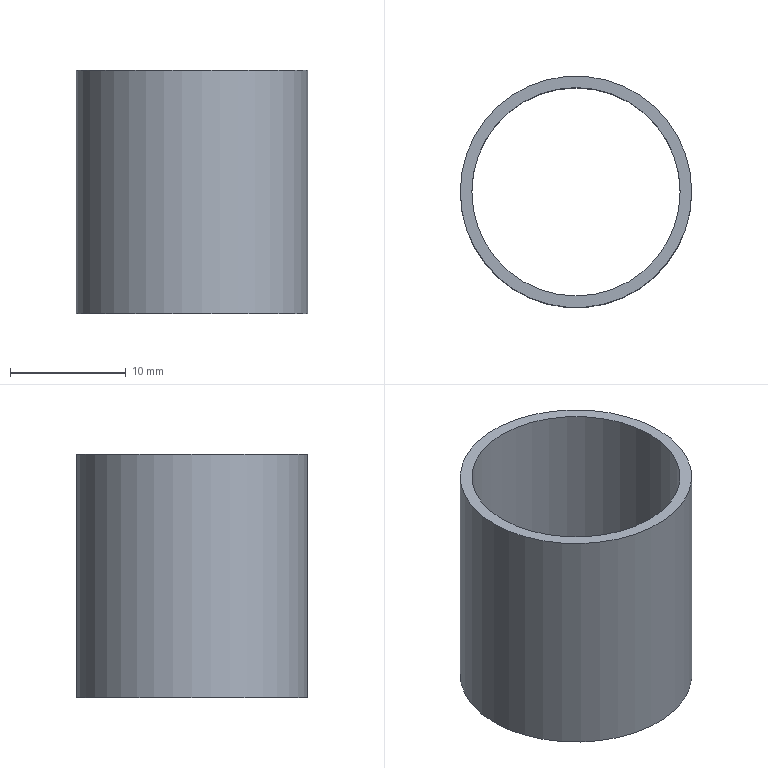Component | NX | 7_2 | 1 solid | 4 faces | box 20 x 20 x 21 mm | volume 1253 mm3 | cylinder 2 | plane 2 | commonest cylinder face diameters 20 x1 18 x1
STEP:
#1=CARTESIAN_POINT('',(0.,0.,0.));
#2=DIRECTION('',(0.,0.,1.));
#3=DIRECTION('',(1.,0.,0.));
#4=AXIS2_PLACEMENT_3D('',#1,#2,#3);
#5=CARTESIAN_POINT('',(10.,-16.5,29.));
#6=VERTEX_POINT('',#5);
#7=CARTESIAN_POINT('',(-0.0000016,-16.5,29.));
#8=DIRECTION('',(0.,0.,1.));
#9=DIRECTION('',(1.,0.00000005,0.));
#10=AXIS2_PLACEMENT_3D('',#7,#8,#9);
#11=CIRCLE('',#10,10.);
#12=CARTESIAN_POINT('',(-0.0000016,-16.5,29.));
#13=DIRECTION('',(0.,0.,-1.));
#14=DIRECTION('',(-1.,-0.00000005,0.));
#15=AXIS2_PLACEMENT_3D('',#12,#13,#14);
#16=CYLINDRICAL_SURFACE('',#15,10.);
#17=CARTESIAN_POINT('',(9.425,0.));
#18=DIRECTION('',(-1.,0.));
#19=VECTOR('',#18,1.);
#20=LINE('',#17,#19);
#21=(GEOMETRIC_REPRESENTATION_CONTEXT(2)PARAMETRIC_REPRESENTATION_CONTEXT()REPRESENTATION_CONTEXT('',''));
#22=DEFINITIONAL_REPRESENTATION('',(#20),#21);
#23=PCURVE('',#16,#22);
#24=CARTESIAN_POINT('',(-0.0000016,-16.5,29.));
#25=DIRECTION('',(0.,0.,1.));
#26=DIRECTION('',(1.,0.00000005,0.));
#27=AXIS2_PLACEMENT_3D('',#24,#25,#26);
#28=PLANE('',#27);
#29=CARTESIAN_POINT('',(0.,0.));
#30=DIRECTION('',(1.,0.));
#31=AXIS2_PLACEMENT_2D('',#29,#30);
#32=CIRCLE('',#31,10.);
#33=(GEOMETRIC_REPRESENTATION_CONTEXT(2)PARAMETRIC_REPRESENTATION_CONTEXT()REPRESENTATION_CONTEXT('',''));
#34=DEFINITIONAL_REPRESENTATION('',(#32),#33);
#35=PCURVE('',#28,#34);
#36=SURFACE_CURVE('',#11,(#23,#35),.PCURVE_S1.);
#37=EDGE_CURVE('',#6,#6,#36,.T.);
#38=ORIENTED_EDGE('',*,*,#37,.F.);
#39=CARTESIAN_POINT('',(10.,-16.5,8.));
#40=VERTEX_POINT('',#39);
#41=CARTESIAN_POINT('',(10.,-16.5,29.));
#42=CARTESIAN_POINT('',(10.,-16.5,8.));
#43=B_SPLINE_CURVE_WITH_KNOTS('',1,(#41,#42),.UNSPECIFIED.,.F.,.F.,(2,2),(0.,21.),.PIECEWISE_BEZIER_KNOTS.);
#44=CARTESIAN_POINT('',(9.425,0.));
#45=DIRECTION('',(0.,1.));
#46=VECTOR('',#45,1.);
#47=LINE('',#44,#46);
#48=(GEOMETRIC_REPRESENTATION_CONTEXT(2)PARAMETRIC_REPRESENTATION_CONTEXT()REPRESENTATION_CONTEXT('',''));
#49=DEFINITIONAL_REPRESENTATION('',(#47),#48);
#50=PCURVE('',#16,#49);
#51=CARTESIAN_POINT('',(3.142,0.));
#52=DIRECTION('',(0.,1.));
#53=VECTOR('',#52,1.);
#54=LINE('',#51,#53);
#55=(GEOMETRIC_REPRESENTATION_CONTEXT(2)PARAMETRIC_REPRESENTATION_CONTEXT()REPRESENTATION_CONTEXT('',''));
#56=DEFINITIONAL_REPRESENTATION('',(#54),#55);
#57=PCURVE('',#16,#56);
#58=SEAM_CURVE('',#43,(#50,#57),.PCURVE_S1.);
#59=EDGE_CURVE('',#6,#40,#58,.T.);
#60=ORIENTED_EDGE('',*,*,#59,.T.);
#61=CARTESIAN_POINT('',(-0.0000016,-16.5,8.));
#62=DIRECTION('',(0.,0.,1.));
#63=DIRECTION('',(1.,0.00000005,0.));
#64=AXIS2_PLACEMENT_3D('',#61,#62,#63);
#65=CIRCLE('',#64,10.);
#66=CARTESIAN_POINT('',(9.425,21.));
#67=DIRECTION('',(-1.,0.));
#68=VECTOR('',#67,1.);
#69=LINE('',#66,#68);
#70=(GEOMETRIC_REPRESENTATION_CONTEXT(2)PARAMETRIC_REPRESENTATION_CONTEXT()REPRESENTATION_CONTEXT('',''));
#71=DEFINITIONAL_REPRESENTATION('',(#69),#70);
#72=PCURVE('',#16,#71);
#73=CARTESIAN_POINT('',(-0.0000016,-16.5,8.));
#74=DIRECTION('',(0.,0.,1.));
#75=DIRECTION('',(1.,0.00000005,0.));
#76=AXIS2_PLACEMENT_3D('',#73,#74,#75);
#77=PLANE('',#76);
#78=CARTESIAN_POINT('',(0.,0.));
#79=DIRECTION('',(1.,0.));
#80=AXIS2_PLACEMENT_2D('',#78,#79);
#81=CIRCLE('',#80,10.);
#82=(GEOMETRIC_REPRESENTATION_CONTEXT(2)PARAMETRIC_REPRESENTATION_CONTEXT()REPRESENTATION_CONTEXT('',''));
#83=DEFINITIONAL_REPRESENTATION('',(#81),#82);
#84=PCURVE('',#77,#83);
#85=SURFACE_CURVE('',#65,(#72,#84),.PCURVE_S1.);
#86=EDGE_CURVE('',#40,#40,#85,.T.);
#87=ORIENTED_EDGE('',*,*,#86,.T.);
#88=ORIENTED_EDGE('',*,*,#59,.F.);
#89=EDGE_LOOP('',(#38,#60,#87,#88));
#90=FACE_BOUND('',#89,.T.);
#91=ADVANCED_FACE('',(#90),#16,.T.);
#92=CARTESIAN_POINT('',(9.,-16.5,29.));
#93=VERTEX_POINT('',#92);
#94=CARTESIAN_POINT('',(-0.0000016,-16.5,29.));
#95=DIRECTION('',(0.,0.,1.));
#96=DIRECTION('',(1.,0.00000005,0.));
#97=AXIS2_PLACEMENT_3D('',#94,#95,#96);
#98=CIRCLE('',#97,9.);
#99=CARTESIAN_POINT('',(-0.0000016,-16.5,29.));
#100=DIRECTION('',(0.,0.,-1.));
#101=DIRECTION('',(-1.,-0.00000005,0.));
#102=AXIS2_PLACEMENT_3D('',#99,#100,#101);
#103=CYLINDRICAL_SURFACE('',#102,9.);
#104=CARTESIAN_POINT('',(9.425,0.));
#105=DIRECTION('',(-1.,0.));
#106=VECTOR('',#105,1.);
#107=LINE('',#104,#106);
#108=(GEOMETRIC_REPRESENTATION_CONTEXT(2)PARAMETRIC_REPRESENTATION_CONTEXT()REPRESENTATION_CONTEXT('',''));
#109=DEFINITIONAL_REPRESENTATION('',(#107),#108);
#110=PCURVE('',#103,#109);
#111=CARTESIAN_POINT('',(0.,0.));
#112=DIRECTION('',(1.,-0.));
#113=AXIS2_PLACEMENT_2D('',#111,#112);
#114=CIRCLE('',#113,9.);
#115=(GEOMETRIC_REPRESENTATION_CONTEXT(2)PARAMETRIC_REPRESENTATION_CONTEXT()REPRESENTATION_CONTEXT('',''));
#116=DEFINITIONAL_REPRESENTATION('',(#114),#115);
#117=PCURVE('',#28,#116);
#118=SURFACE_CURVE('',#98,(#110,#117),.PCURVE_S1.);
#119=EDGE_CURVE('',#93,#93,#118,.T.);
#120=ORIENTED_EDGE('',*,*,#119,.F.);
#121=CARTESIAN_POINT('',(9.,-16.5,8.));
#122=VERTEX_POINT('',#121);
#123=CARTESIAN_POINT('',(9.,-16.5,29.));
#124=CARTESIAN_POINT('',(9.,-16.5,8.));
#125=B_SPLINE_CURVE_WITH_KNOTS('',1,(#123,#124),.UNSPECIFIED.,.F.,.F.,(2,2),(0.,21.),.PIECEWISE_BEZIER_KNOTS.);
#126=CARTESIAN_POINT('',(9.425,0.));
#127=DIRECTION('',(0.,1.));
#128=VECTOR('',#127,1.);
#129=LINE('',#126,#128);
#130=(GEOMETRIC_REPRESENTATION_CONTEXT(2)PARAMETRIC_REPRESENTATION_CONTEXT()REPRESENTATION_CONTEXT('',''));
#131=DEFINITIONAL_REPRESENTATION('',(#129),#130);
#132=PCURVE('',#103,#131);
#133=CARTESIAN_POINT('',(3.142,0.));
#134=DIRECTION('',(0.,1.));
#135=VECTOR('',#134,1.);
#136=LINE('',#133,#135);
#137=(GEOMETRIC_REPRESENTATION_CONTEXT(2)PARAMETRIC_REPRESENTATION_CONTEXT()REPRESENTATION_CONTEXT('',''));
#138=DEFINITIONAL_REPRESENTATION('',(#136),#137);
#139=PCURVE('',#103,#138);
#140=SEAM_CURVE('',#125,(#132,#139),.PCURVE_S1.);
#141=EDGE_CURVE('',#93,#122,#140,.T.);
#142=ORIENTED_EDGE('',*,*,#141,.T.);
#143=CARTESIAN_POINT('',(-0.0000016,-16.5,8.));
#144=DIRECTION('',(0.,0.,1.));
#145=DIRECTION('',(1.,0.00000005,0.));
#146=AXIS2_PLACEMENT_3D('',#143,#144,#145);
#147=CIRCLE('',#146,9.);
#148=CARTESIAN_POINT('',(9.425,21.));
#149=DIRECTION('',(-1.,0.));
#150=VECTOR('',#149,1.);
#151=LINE('',#148,#150);
#152=(GEOMETRIC_REPRESENTATION_CONTEXT(2)PARAMETRIC_REPRESENTATION_CONTEXT()REPRESENTATION_CONTEXT('',''));
#153=DEFINITIONAL_REPRESENTATION('',(#151),#152);
#154=PCURVE('',#103,#153);
#155=CARTESIAN_POINT('',(0.,0.));
#156=DIRECTION('',(1.,-0.));
#157=AXIS2_PLACEMENT_2D('',#155,#156);
#158=CIRCLE('',#157,9.);
#159=(GEOMETRIC_REPRESENTATION_CONTEXT(2)PARAMETRIC_REPRESENTATION_CONTEXT()REPRESENTATION_CONTEXT('',''));
#160=DEFINITIONAL_REPRESENTATION('',(#158),#159);
#161=PCURVE('',#77,#160);
#162=SURFACE_CURVE('',#147,(#154,#161),.PCURVE_S1.);
#163=EDGE_CURVE('',#122,#122,#162,.T.);
#164=ORIENTED_EDGE('',*,*,#163,.T.);
#165=ORIENTED_EDGE('',*,*,#141,.F.);
#166=EDGE_LOOP('',(#120,#142,#164,#165));
#167=FACE_BOUND('',#166,.F.);
#168=ADVANCED_FACE('',(#167),#103,.F.);
#169=ORIENTED_EDGE('',*,*,#37,.T.);
#170=EDGE_LOOP('',(#169));
#171=FACE_BOUND('',#170,.T.);
#172=ORIENTED_EDGE('',*,*,#119,.F.);
#173=EDGE_LOOP('',(#172));
#174=FACE_BOUND('',#173,.T.);
#175=ADVANCED_FACE('',(#171,#174),#28,.T.);
#176=ORIENTED_EDGE('',*,*,#86,.F.);
#177=EDGE_LOOP('',(#176));
#178=FACE_BOUND('',#177,.T.);
#179=ORIENTED_EDGE('',*,*,#163,.T.);
#180=EDGE_LOOP('',(#179));
#181=FACE_BOUND('',#180,.T.);
#182=ADVANCED_FACE('',(#178,#181),#77,.F.);
#183=CLOSED_SHELL('',(#91,#168,#175,#182));
#184=MANIFOLD_SOLID_BREP('',#183);
#185=(LENGTH_UNIT()NAMED_UNIT(*)SI_UNIT(.MILLI.,.METRE.));
#186=UNCERTAINTY_MEASURE_WITH_UNIT(LENGTH_MEASURE(0.00001),#185,'','');
#187=(NAMED_UNIT(*)PLANE_ANGLE_UNIT()SI_UNIT($,.RADIAN.));
#188=(NAMED_UNIT(*)SI_UNIT($,.STERADIAN.)SOLID_ANGLE_UNIT());
#189=(GEOMETRIC_REPRESENTATION_CONTEXT(3)GLOBAL_UNCERTAINTY_ASSIGNED_CONTEXT((#186))GLOBAL_UNIT_ASSIGNED_CONTEXT((#185,#187,#188))REPRESENTATION_CONTEXT('',''));
#190=ADVANCED_BREP_SHAPE_REPRESENTATION('',(#4,#184),#189);